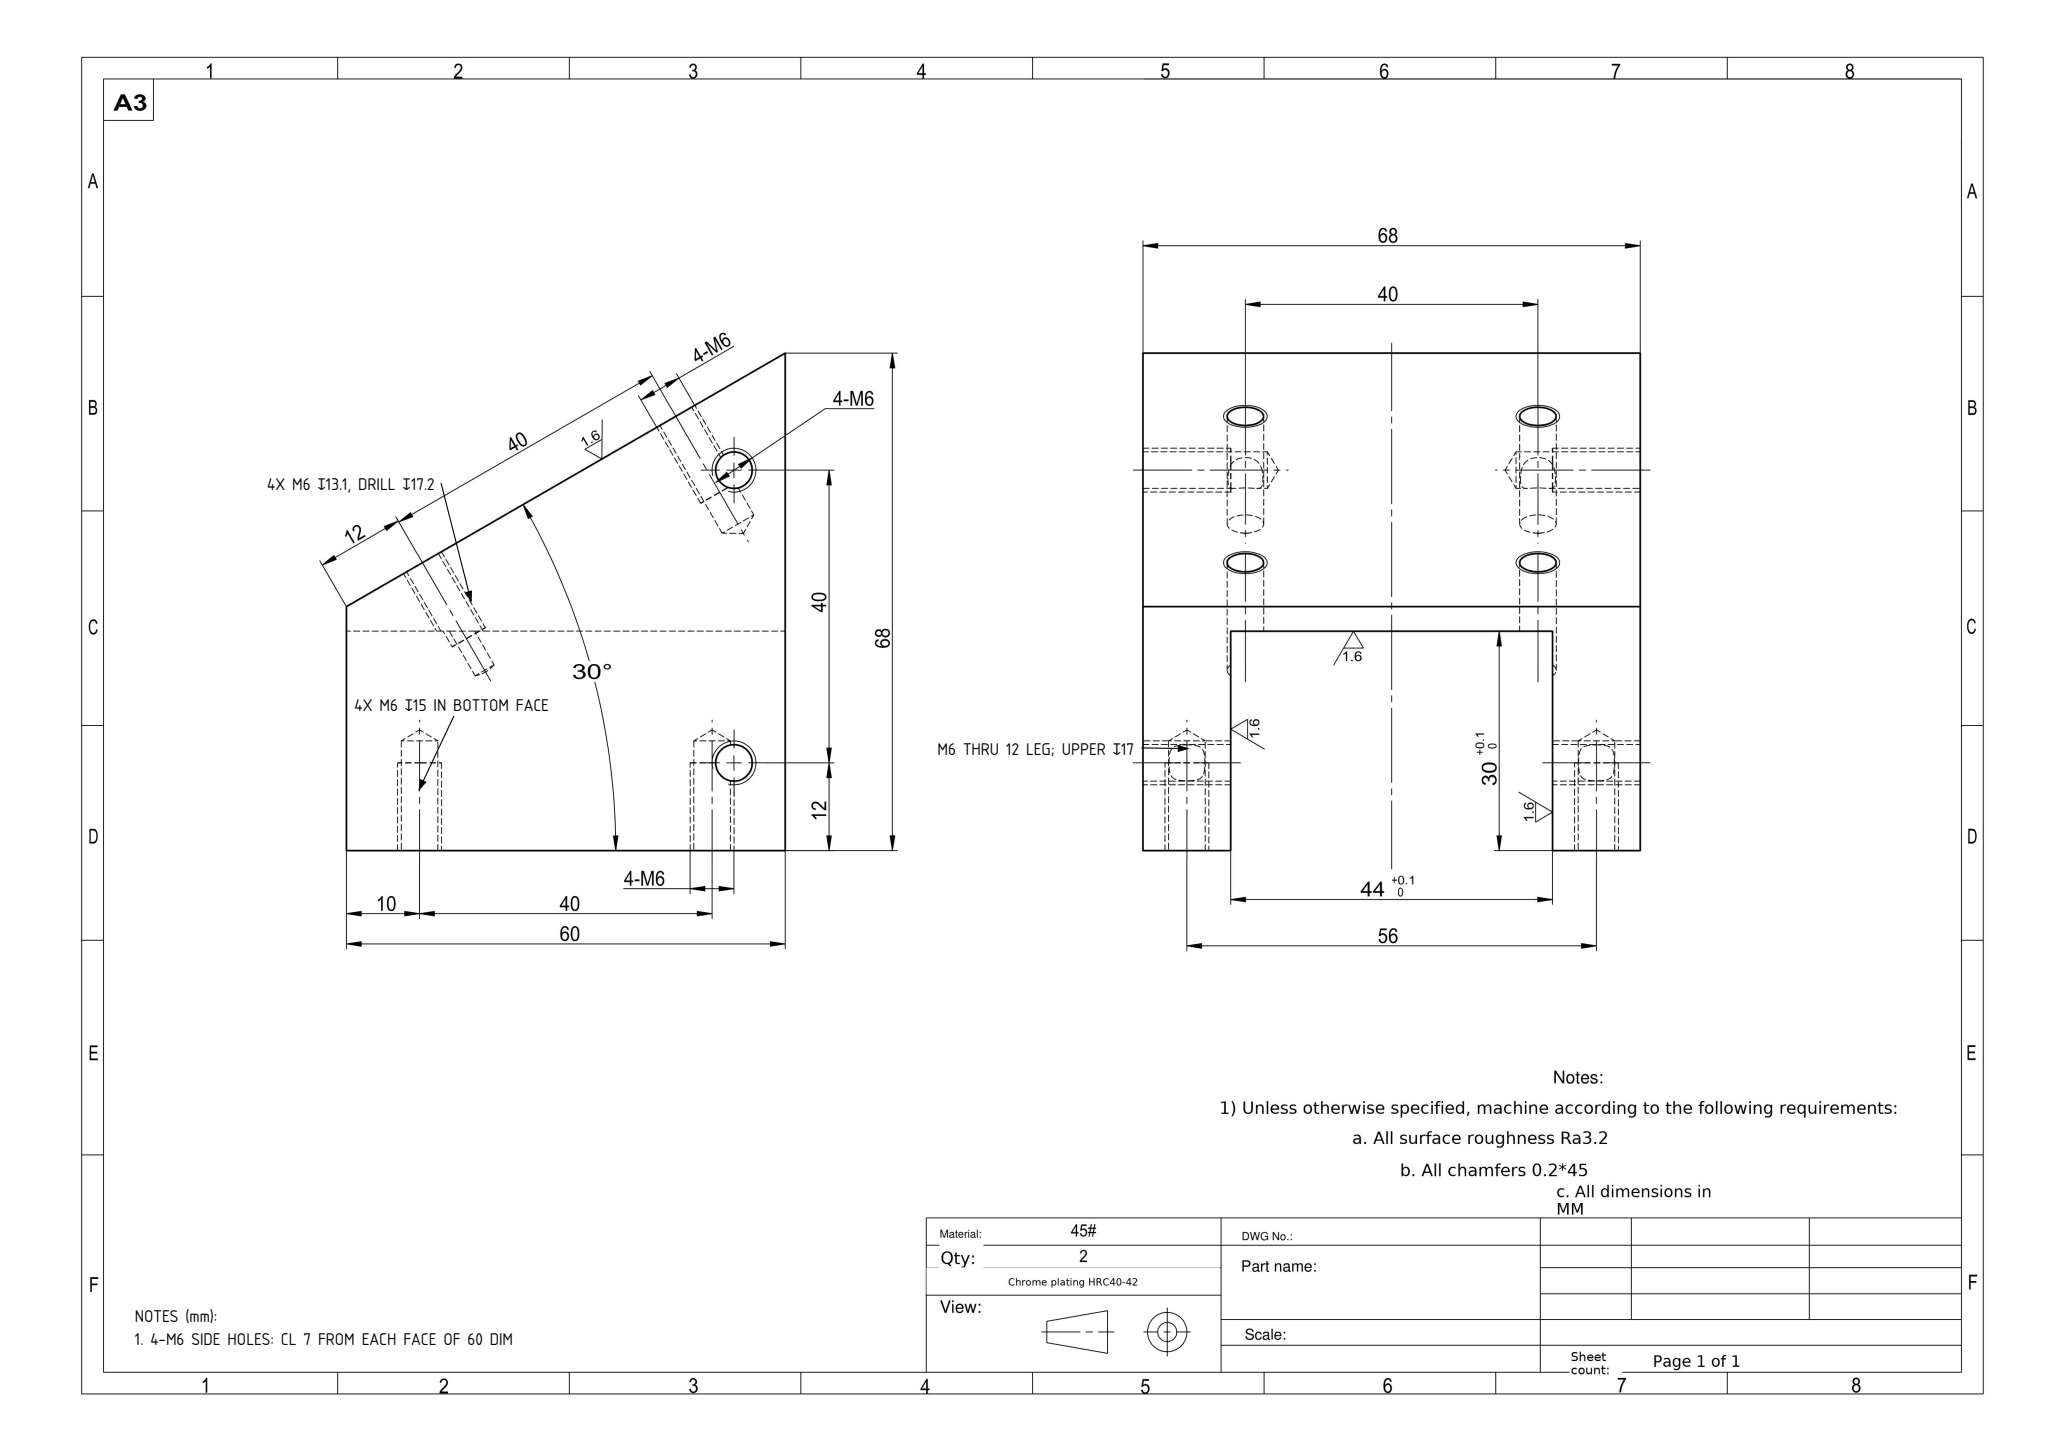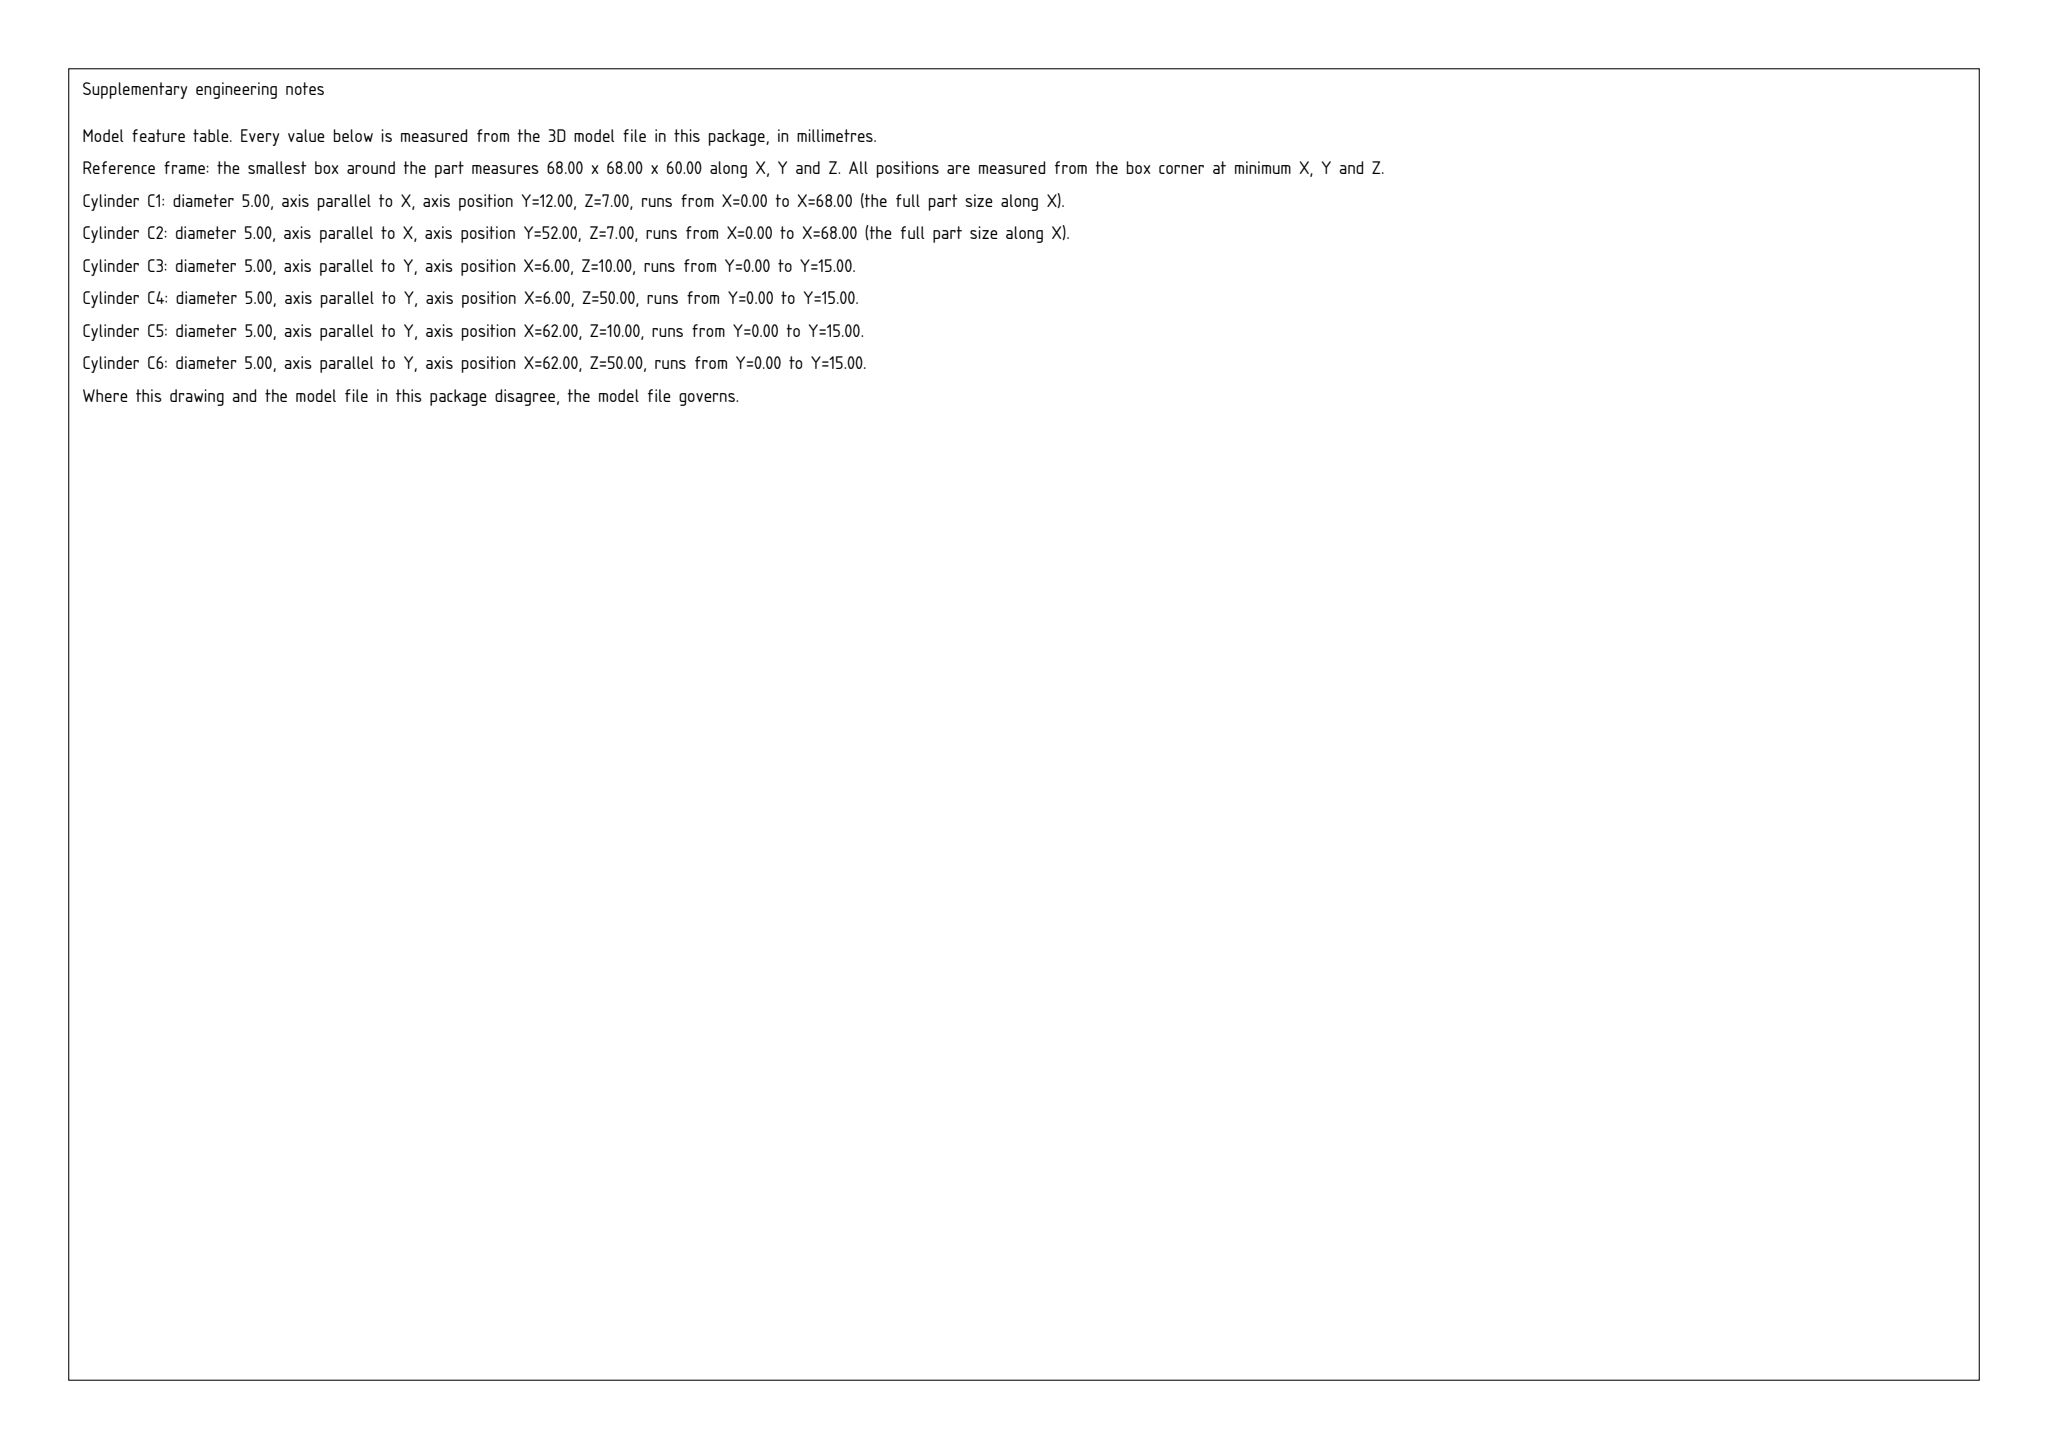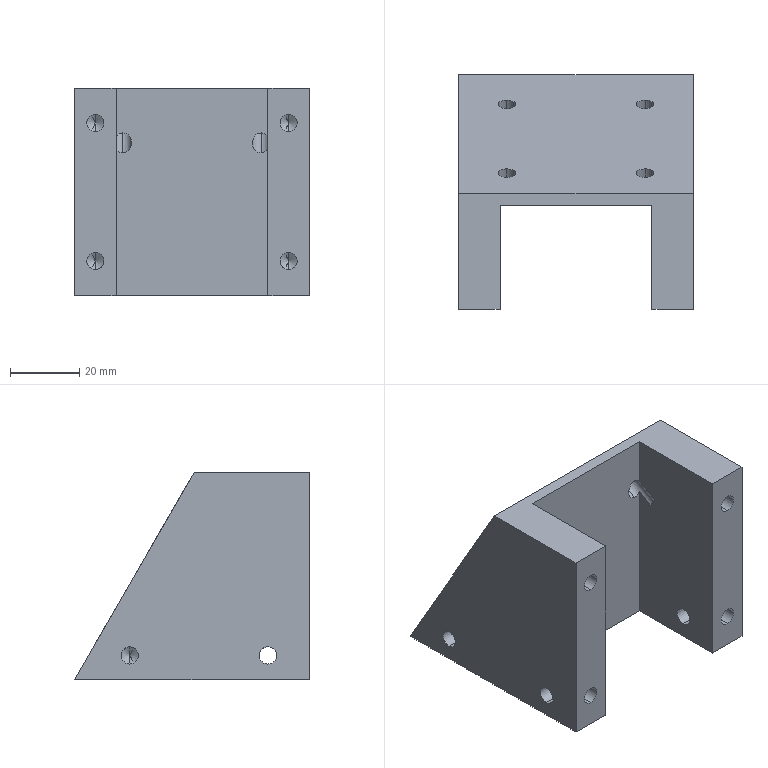Part | SolidWorks | mm | material 45# | 1 solid | 52 faces | box 68 x 68 x 60 mm | volume 124162 mm3 | cylinder 24 | cone 18 | plane 10 | commonest cylinder face diameters 5 x24
Drawing notes:
4-M6 SIDE HOLES: CL 7 FROM EACH FACE OF 60 DIM | from the solid: Ø5 cyls axis x at z=7 (and mirror 53), y=12 & y=52, from 60 bbox
4-M6 DP 15 IN BOTTOM FACE, 4 PLCS | from the solid: Ø5 cyls axis y at (x6,z10),(x6,z50),(x62,z10),(x62,z50), L=15
4-M6 NORM TO 30° FACE: DRILL DP 17.2, TAP DP 13.1 | from the solid: Ø5 cyls at x=14/54, z=14.97 & 49.61, L=17.22 and 13.11
4-M6 SIDE HOLES: LOWER THRU 12 LEG, UPPER DP 17 | from the solid: Ø5 axis x L=12 at y=12 (12 wall) ; Ø5 axis x L=17 at y=52
build123d program:
from build123d import *

# Parameters (mm, degrees)
BOSS_EXTRUDE1_DEPTH        = 34
CUT_EXTRUDE1_DEPTH         = 82.731
CUT_EXTRUDE1_DEPTH_BACK    = 82.731
SKETCH2_W                  = 44
SKETCH2_H                  = 30
M6_TAPPED_HOLE1_D          = 5
M6_TAPPED_HOLE1_DEPTH      = 15
M6_TAPPED_HOLE1_TIP        = 1.502
M6_TAPPED_HOLE2_AT_2_COUNT = 2
M6_TAPPED_HOLE2_AT_2_PITCH = 40
M6_TAPPED_HOLE3_D          = 5
M6_TAPPED_HOLE3_DEPTH      = 17
M6_TAPPED_HOLE3_TIP        = 1.502


with BuildPart() as part:
    # Sketch1 → Boss-Extrude1 (new, symmetric)
    with BuildSketch(Plane(origin=(0, 0, 0), x_dir=(0, 0, -1), z_dir=(1, 0, 0))):
        Polygon((-30, 0), (30, 0), (30, 68), (-30, 33.359), align=None)
    extrude(amount=BOSS_EXTRUDE1_DEPTH, both=True)

    # Sketch2 → Cut-Extrude1 (cut, two sides: drawn at the far end of the back side and taken through both)
    with BuildSketch(Plane.XY.offset(-CUT_EXTRUDE1_DEPTH_BACK)):
        with Locations((0, 15)):
            Rectangle(SKETCH2_W, SKETCH2_H)
    extrude(amount=CUT_EXTRUDE1_DEPTH + CUT_EXTRUDE1_DEPTH_BACK, mode=Mode.SUBTRACT)

    # M6 Tapped Hole1
    with Locations(Plane(origin=(0, 0, 0), x_dir=(-1, 0, 0), z_dir=(0, -1, 0))):
        with Locations((28, 20), (28, -20), (-28, -20), (-28, 20)):
            Hole(M6_TAPPED_HOLE1_D / 2, depth=M6_TAPPED_HOLE1_DEPTH)
            with Locations((0, 0, -(M6_TAPPED_HOLE1_DEPTH + M6_TAPPED_HOLE1_TIP / 2))):  # 118° drill point
                Cone(0, M6_TAPPED_HOLE1_D / 2, M6_TAPPED_HOLE1_TIP, mode=Mode.SUBTRACT)

    # Sketch6 → M6 Tapped Hole2 (revolve, cut)
    with BuildSketch(Plane(origin=(-34, 12, -23), x_dir=(0, 0, 1), z_dir=(0, 1, 0))):
        Polygon((0, 0), (0, 18.502), (2.5, 17), (2.5, 0), align=None)
    m6_tapped_hole2 = revolve(axis=Axis((-40.35, 12, -23), (1, 0, 0)), mode=Mode.SUBTRACT)

    # M6 Tapped Hole2 at 2: M6 Tapped Hole2 ×2
    with Locations(*[(0, i * M6_TAPPED_HOLE2_AT_2_PITCH, 0) for i in range(1, M6_TAPPED_HOLE2_AT_2_COUNT)]):
        add(m6_tapped_hole2, mode=Mode.SUBTRACT)

    # Mirror1: M6 Tapped Hole2 across plane
    add(m6_tapped_hole2.mirror(Plane(origin=(0, 0, 0), x_dir=(0, 0, 1), z_dir=(1, 0, 0))), mode=Mode.SUBTRACT)

    # Mirror1 copy 1 sketch → Mirror1 copy 1 (revolve, cut)
    with BuildSketch(Plane(origin=(34, 52, -23), x_dir=(0, 0, 1), z_dir=(0, 1, 0))):
        Polygon((0, 0), (0, -18.502), (2.5, -17), (2.5, 0), align=None)
    revolve(axis=Axis((40.35, 52, -23), (1, 0, 0)), mode=Mode.SUBTRACT)

    # M6 Tapped Hole3
    with Locations(Plane(origin=(0, 38.01, 21.945), x_dir=(1, 0, 0), z_dir=(0, 0.866, 0.5))):
        with Locations((-20, 2.699), (-20, 42.699), (20, 42.699), (20, 2.699)):
            Hole(M6_TAPPED_HOLE3_D / 2, depth=M6_TAPPED_HOLE3_DEPTH)
            with Locations((0, 0, -(M6_TAPPED_HOLE3_DEPTH + M6_TAPPED_HOLE3_TIP / 2))):  # 118° drill point
                Cone(0, M6_TAPPED_HOLE3_D / 2, M6_TAPPED_HOLE3_TIP, mode=Mode.SUBTRACT)


solid = part.part